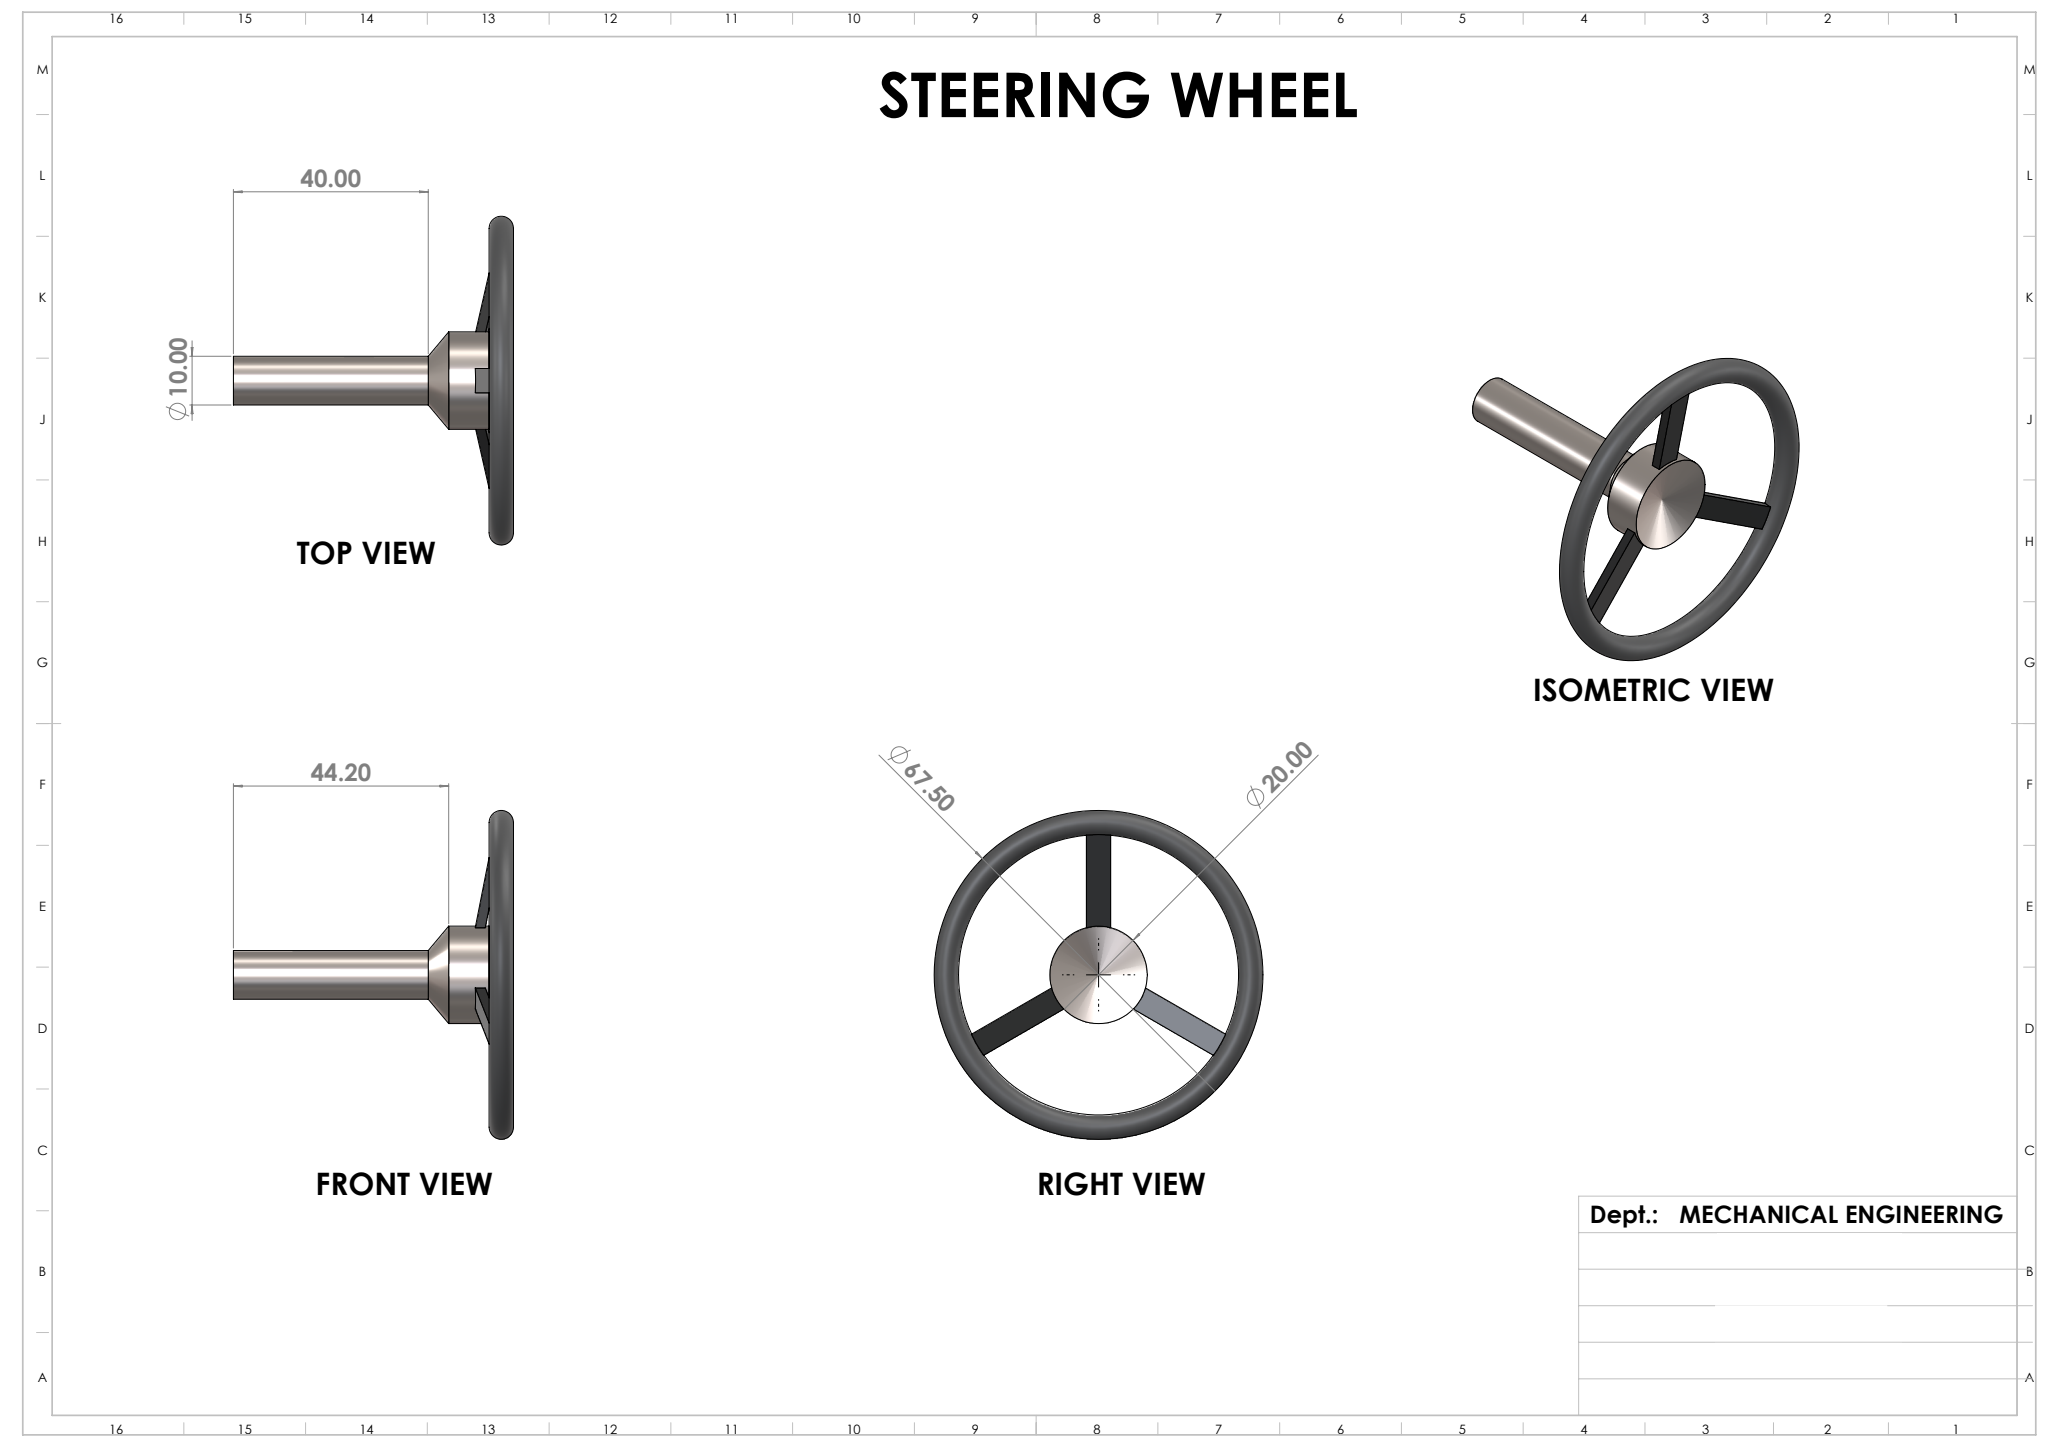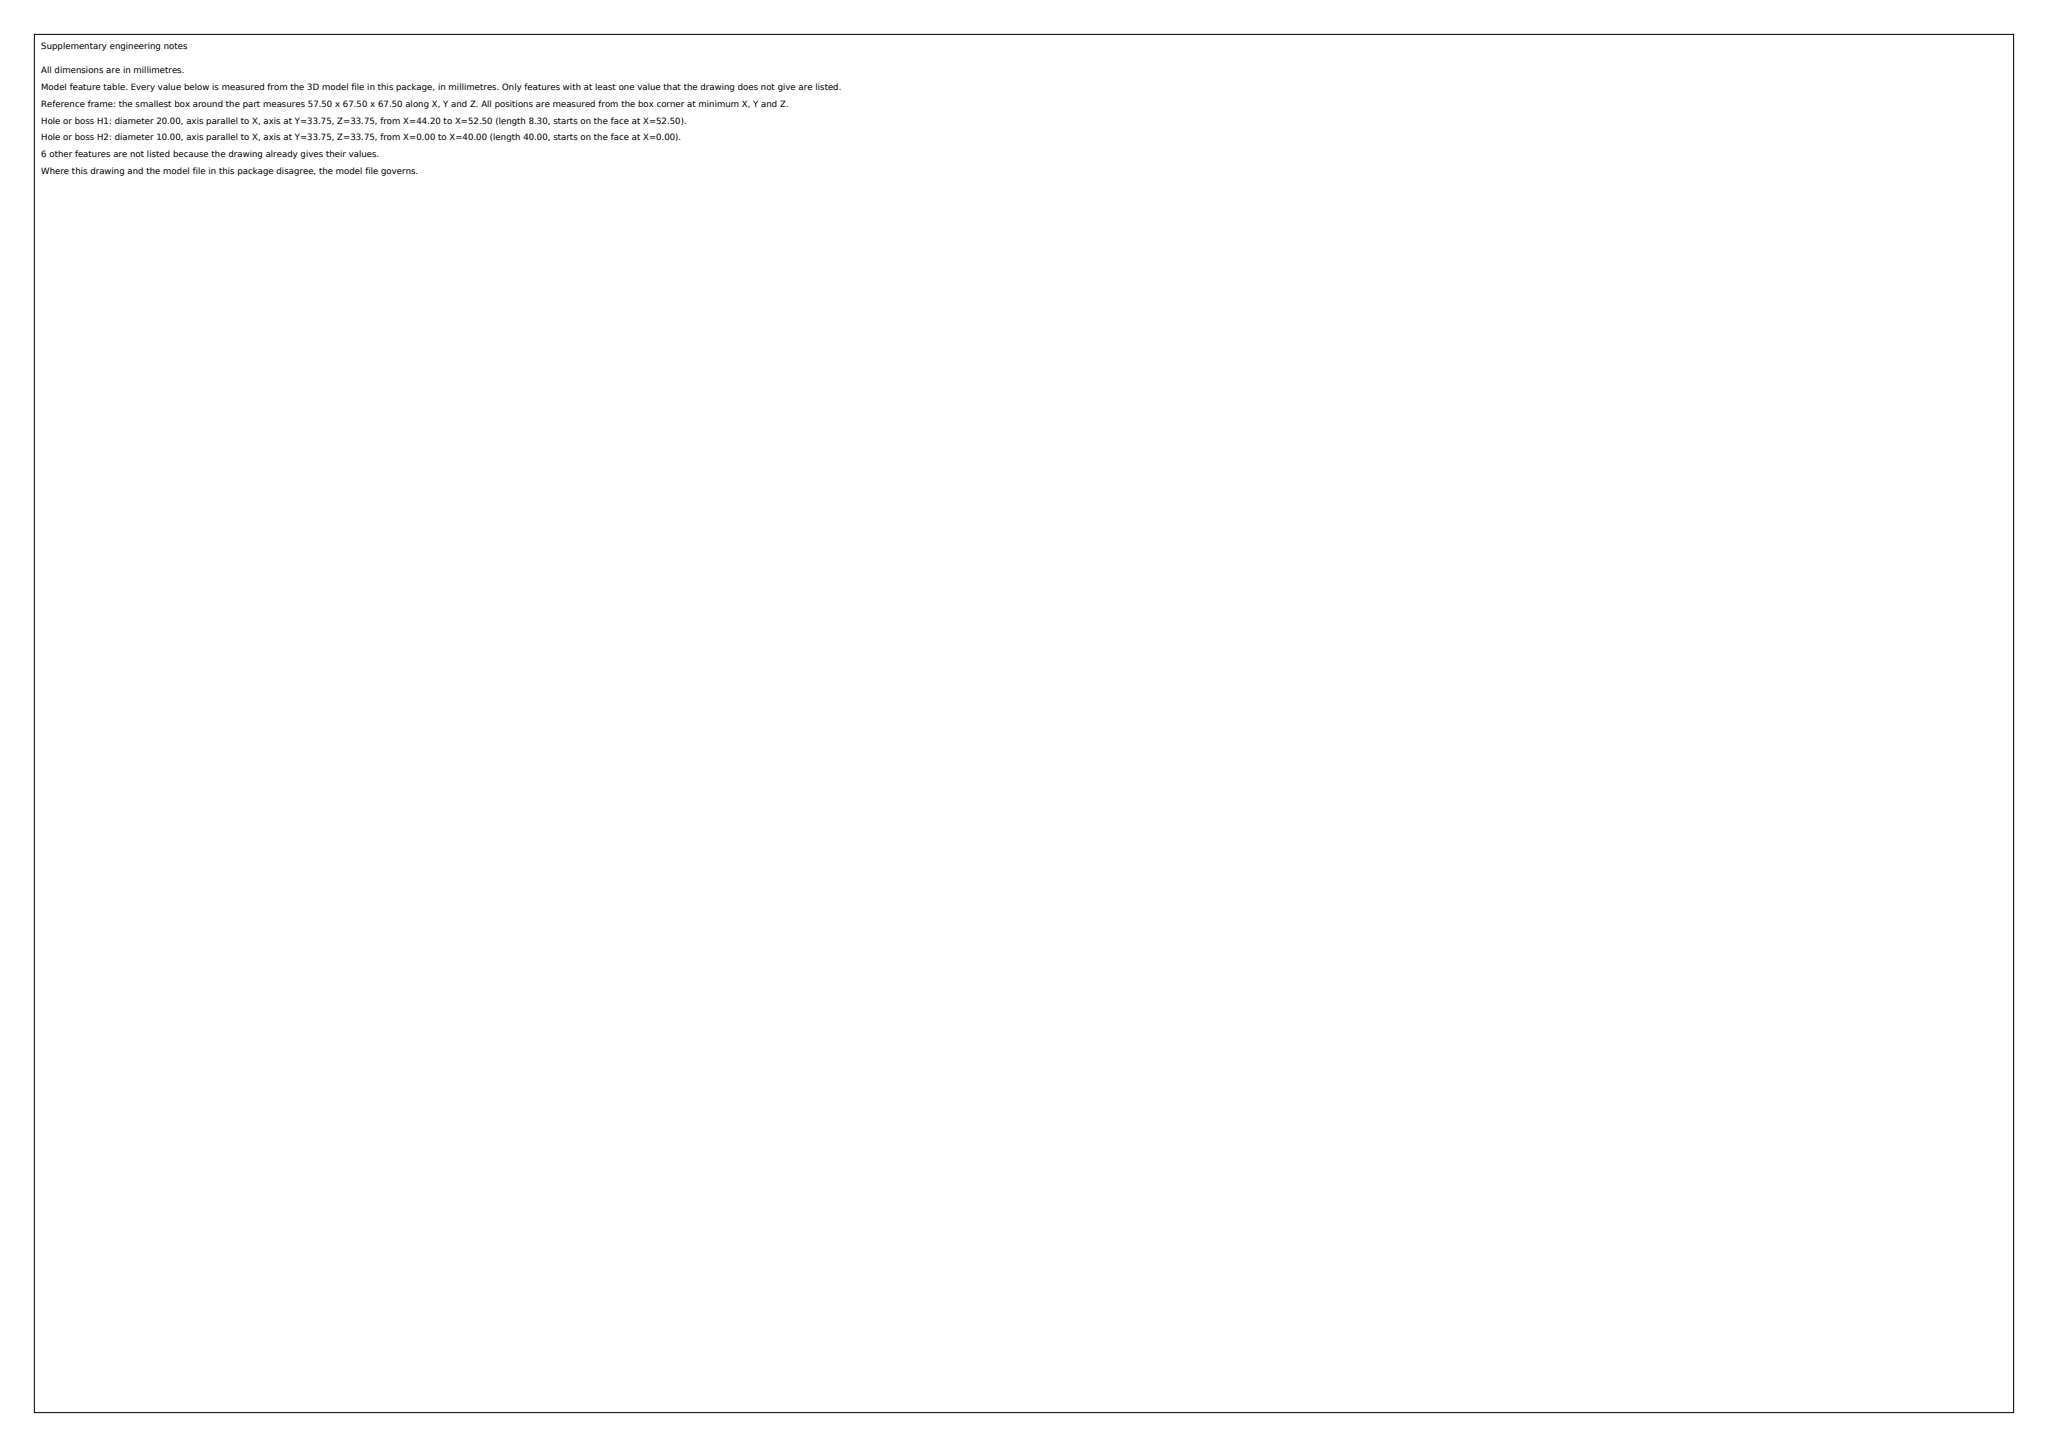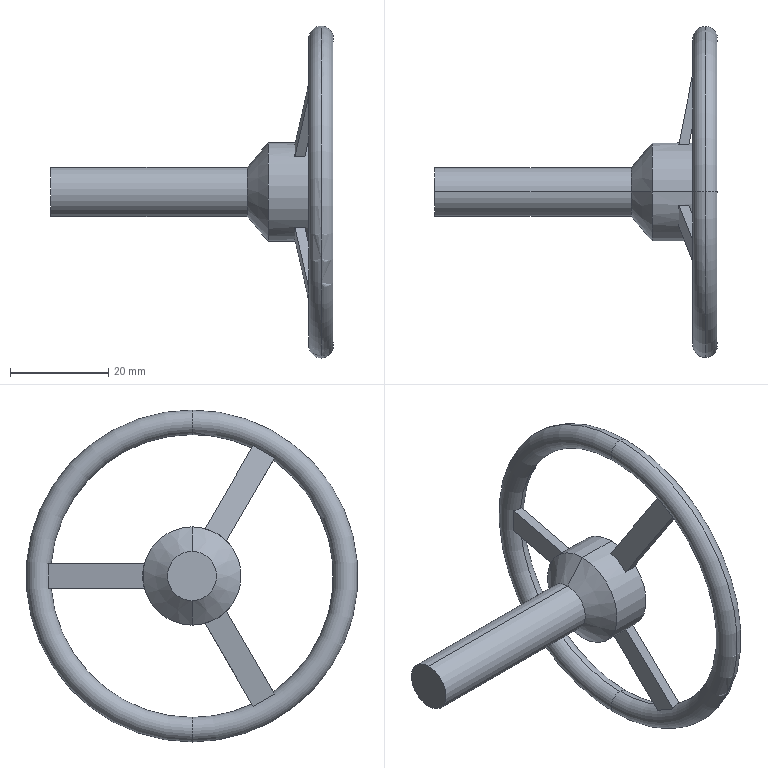Part | SolidWorks | mm | 1 solid | 25 faces | box 57.5 x 67.5 x 67.5 mm | volume 10688 mm3 | plane 13 | torus 4 | cone 4 | cylinder 4 | commonest cylinder face diameters 20 x2 10 x2
Drawing notes:
HUB BOSS Ø20.00, 8.30 LONG, COAXIAL WITH Ø10.00 SHAFT (SHAFT AXIS = DATUM A), BUTTED TO END OF 40.00 SHAFT | from the solid: cylinders[dia,axis,pos_other_axes,length]: [20.0,'x',[null,36.53,36.53],8.3] and [10.0,'x',...,40.0]
CONICAL RECESS Ø20.00, 100° INCLUDED ANGLE, 2.53 DEEP, COAXIAL WITH DATUM A IN HUB FACE | from the solid: cones[included_angle,ref_dia]: [100.0, 20.0]
UNSPECIFIED FILLETS R2.50 (4 PLACES) AT SPOKE-TO-HUB AND SPOKE-TO-RIM BLENDS | from the solid: fillet_radii: [2.5, 4]
ALL DIMENSIONS IN MILLIMETRES; OVERALL LENGTH 57.50 ALONG DATUM A (SHAFT AXIS), WHEEL ENVELOPE 73.06 x 73.06 | from the solid: bbox_xyz: [57.5, 73.062, 73.062], units mm
RIM/SPOKE DISH: CONICAL SURFACE, 151.70° INCLUDED ANGLE, APEX ON AND COAXIAL WITH DATUM A (SHAFT AXIS); CONE DEFINES THE RIM AXIAL PROFILE | from the solid: cones[included_angle,ref_dia] = [151.7, 7921.361] (2 faces)
RIM OUTER ENVELOPE Ø73.06 ABOUT DATUM A; Ø67.50 IS THE RIM TUBE CENTRELINE PATH, NOT THE OUTER DIAMETER | from the solid: bbox_xyz = [57.5, 73.062, 73.062], rim axis centred at (y,z)=(36.53,36.53)
3X SPOKES 5.00 WIDE, SIDE FACES AT 34.03 AND 39.03 FROM BBOX MIN (SYMMETRIC ABOUT DATUM A), EQUALLY SPACED 120° | from the solid: axis_planes[z,34.03] and [z,39.03]; cylinders axis pos (36.53,36.53)
CONICAL RECESS Ø20.00, 100° INCLUDED ANGLE, COAXIAL WITH DATUM A, IN HUB FACE AT 48.30 FROM SHAFT END FACE (X=0, DATUM B) | from the solid: cones [100.0, ref_dia 20.0]; cylinders ⌀10.00 L40.0 + ⌀20.00 L8.3 on x axis; axis_plane[x,0.0]
build123d program:
from build123d import *

# Parameters (mm, degrees)
SKETCH2_R           = 2.5
BOSS_EXTRUDE1_DEPTH = 2.5
CIRPATTERN1_COUNT   = 3


with BuildPart() as part:
    # Sketch1 → Revolve1 (revolve)
    with BuildSketch(Plane.XY, mode=Mode.PRIVATE) as revolve1_sk:
        Polygon((49.971, 0), (0, 0), (0, 5), (40, 5), (44.195, 10), (52.495, 10), align=None)
    revolve(revolve1_sk.sketch.rotate(Axis((49.971, 0, 0), (-1, 0, 0)), 90), axis=Axis((49.971, 0, 0), (-1, 0, 0)))



with BuildPart() as body_2:
    # Sketch2 → Revolve2 (revolve)
    with BuildSketch(Plane.XY, mode=Mode.PRIVATE) as revolve2_sk:
        with Locations((55, 31.25)):
            Circle(SKETCH2_R)
    revolve(revolve2_sk.sketch.rotate(Axis((0, 0, 0), (1, 0, 0)), 90), axis=Axis((0, 0, 0), (1, 0, 0)))


with BuildPart() as part_1:
    add(part.part)

    add(body_2.part)  # Boss-Extrude1 merges body 2
    # Sketch3 → Boss-Extrude1 (add, symmetric)
    with BuildSketch(Plane.XY):
        Polygon((56.02, 31.627), (51.6, 9.2), (49.562, 9.2), (53.982, 31.627), align=None)
    boss_extrude1 = extrude(amount=BOSS_EXTRUDE1_DEPTH, both=True)

    # CirPattern1: Boss-Extrude1 ×3 about axis
    cirpattern1_axis = Axis((0, 0, 0), (1, 0, 0))
    for i in range(1, CIRPATTERN1_COUNT):
        add(boss_extrude1.rotate(cirpattern1_axis, i * 360 / CIRPATTERN1_COUNT))


solid = part_1.part